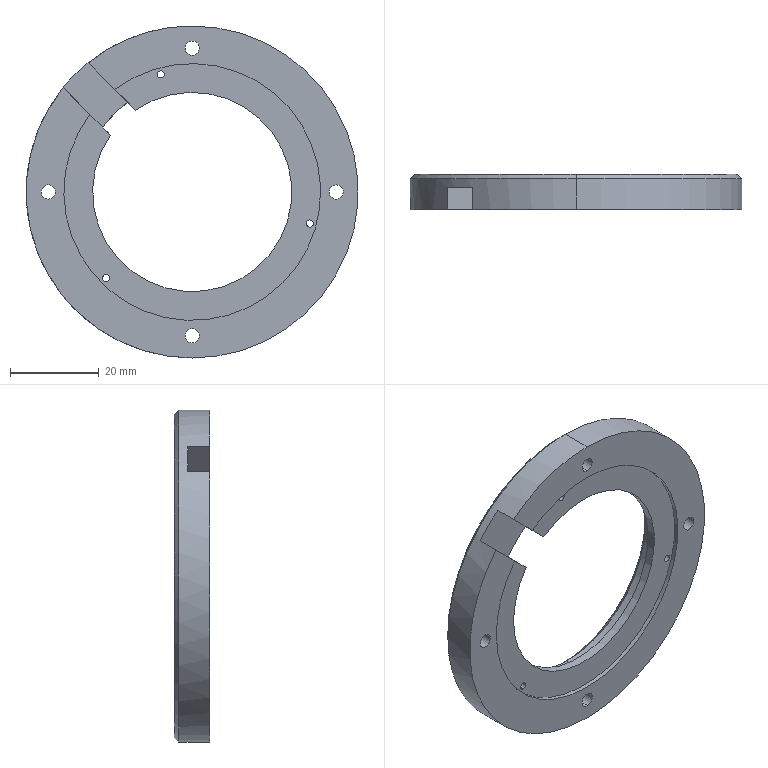CAM job | Mastercam | mm | 4 operations | part box 75 x 8 x 75
1. Contour (Ramp) | 6 - 6 平铣刀
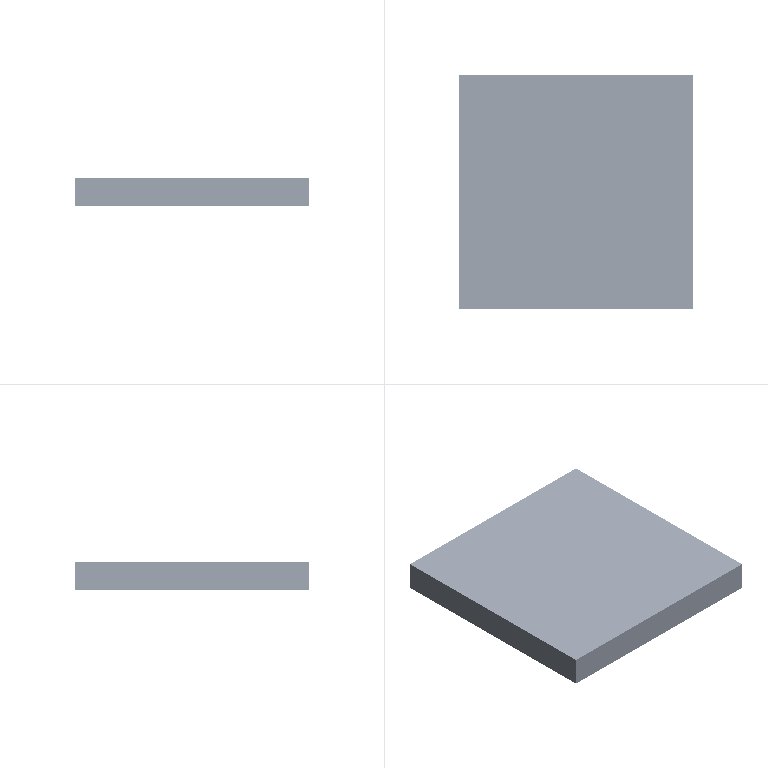2. Contour (2D) | 6 - 6 平铣刀
3. Contour (2D chamfer) | 7 - 4 倒角刀
4. Drill/Counterbore | 1 - 2 倒角刀